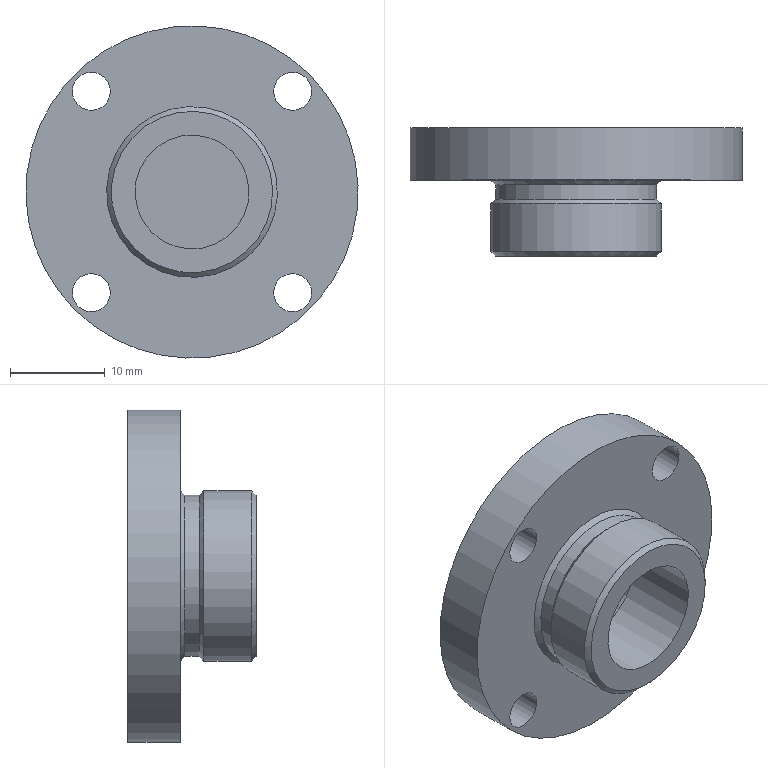Component | NX | CLHKJG_02_SEAL_END_CAP | 1 solid | 19 faces | volume 5564 mm3 | cylinder 10 | plane 6 | cone 3 | commonest cylinder face diameters 4 x4 18 x2 35 x1 17 x1 12 x1 13 x1